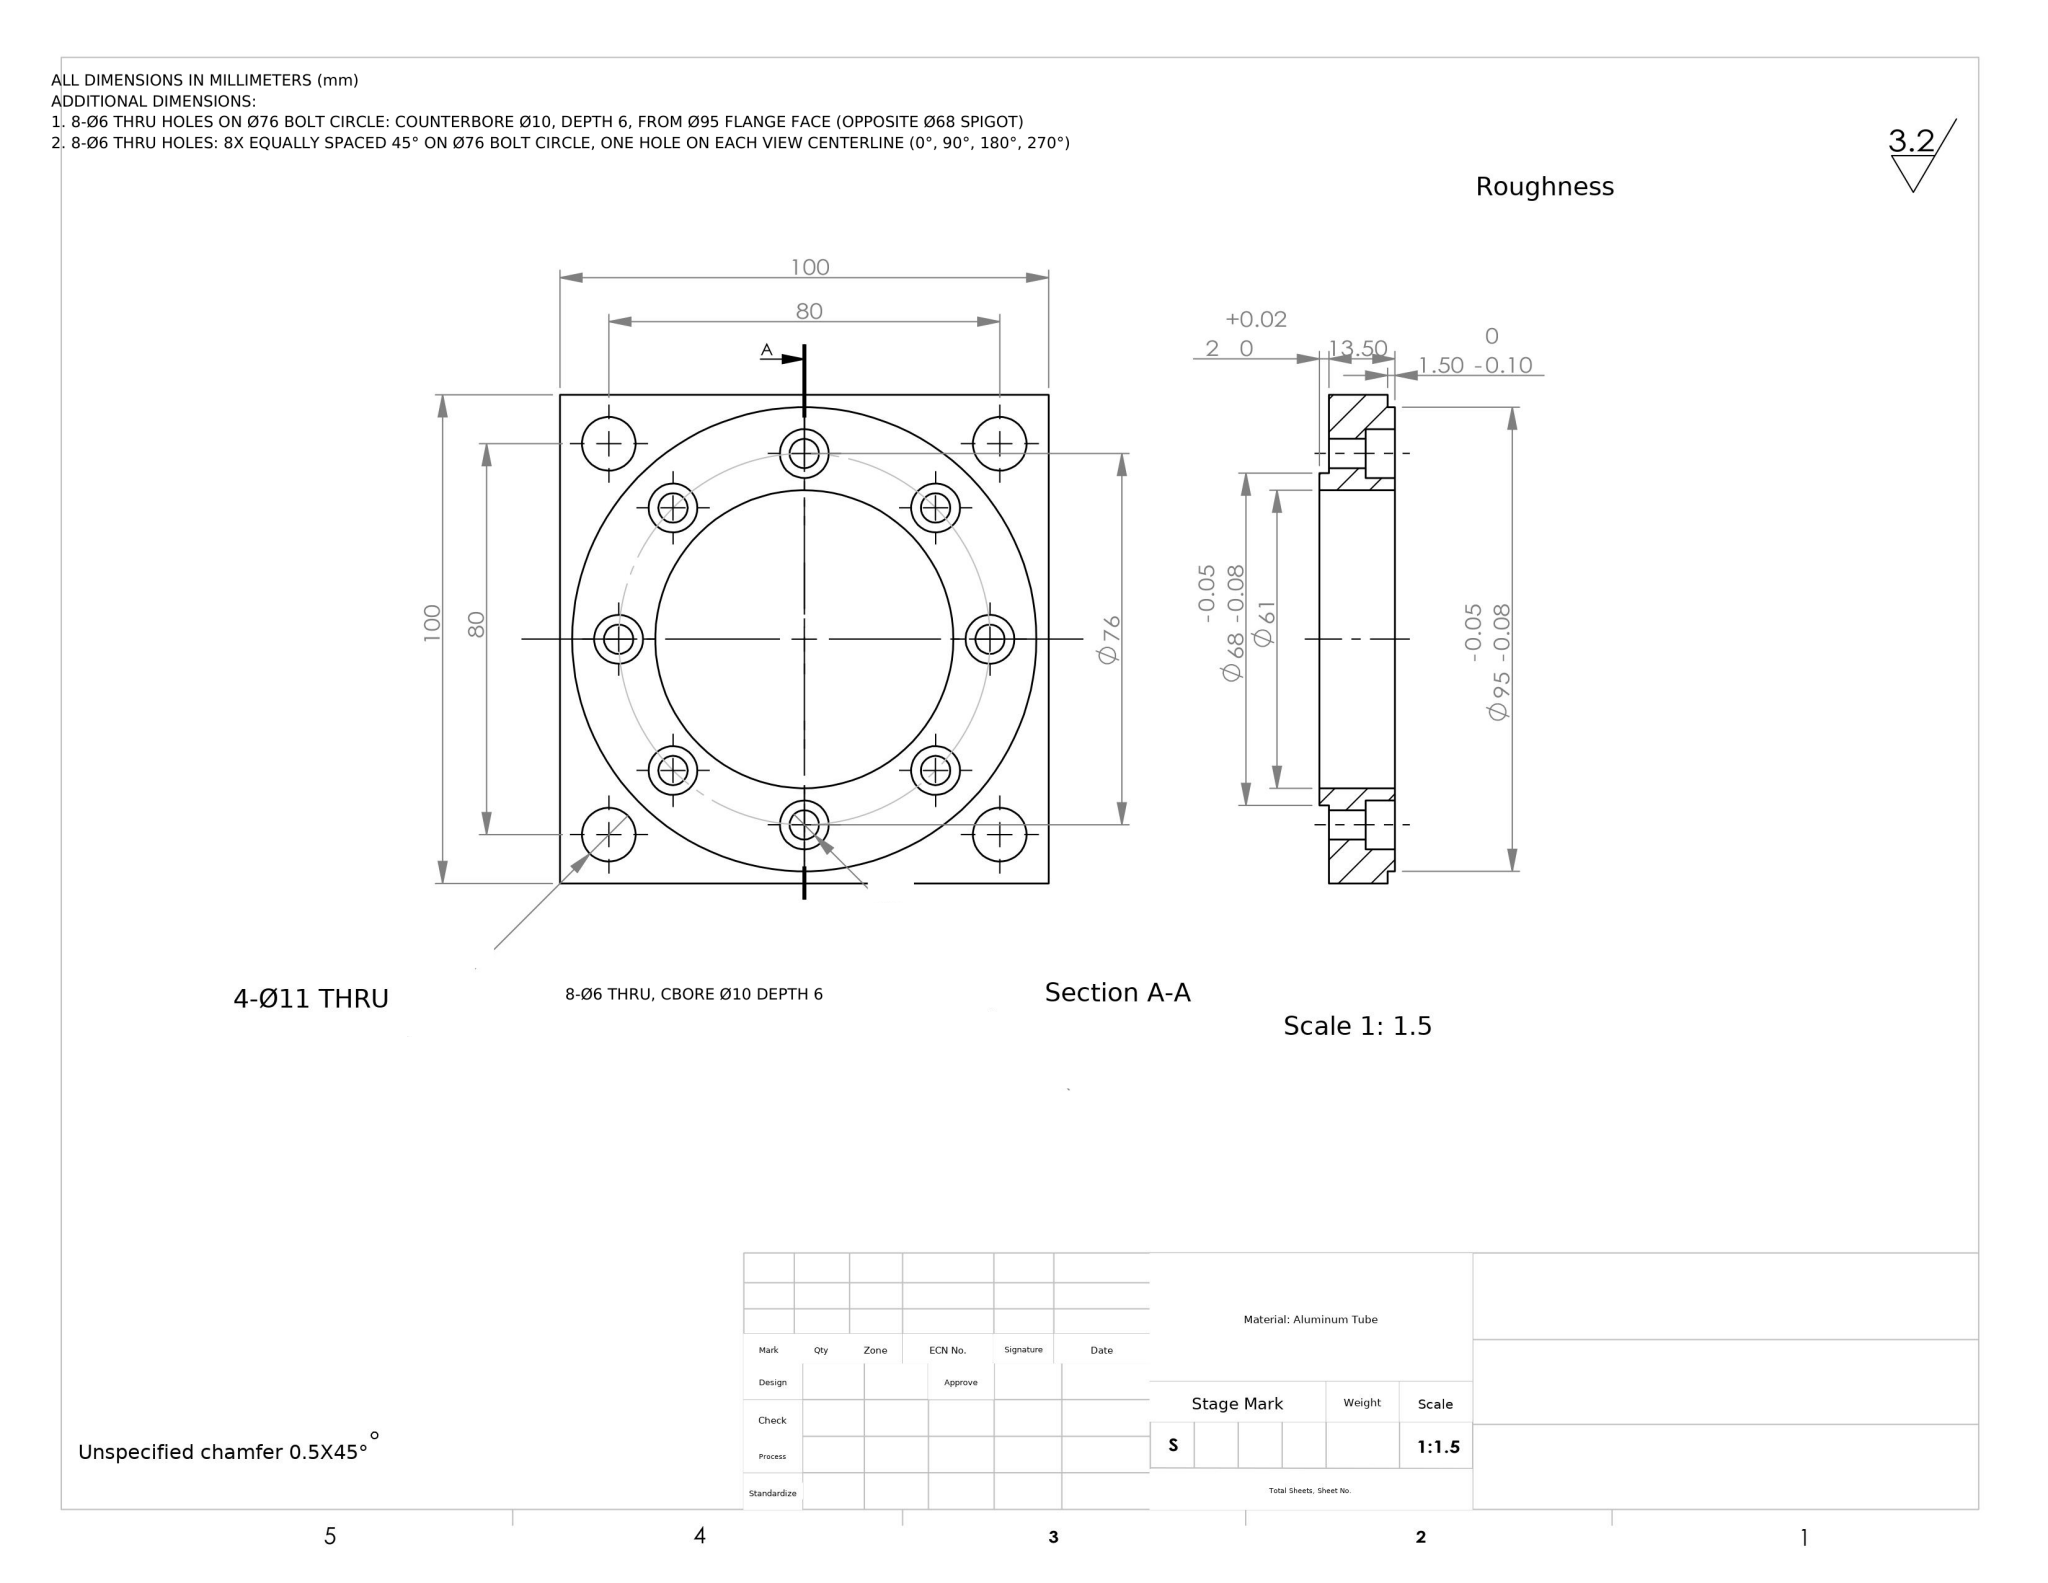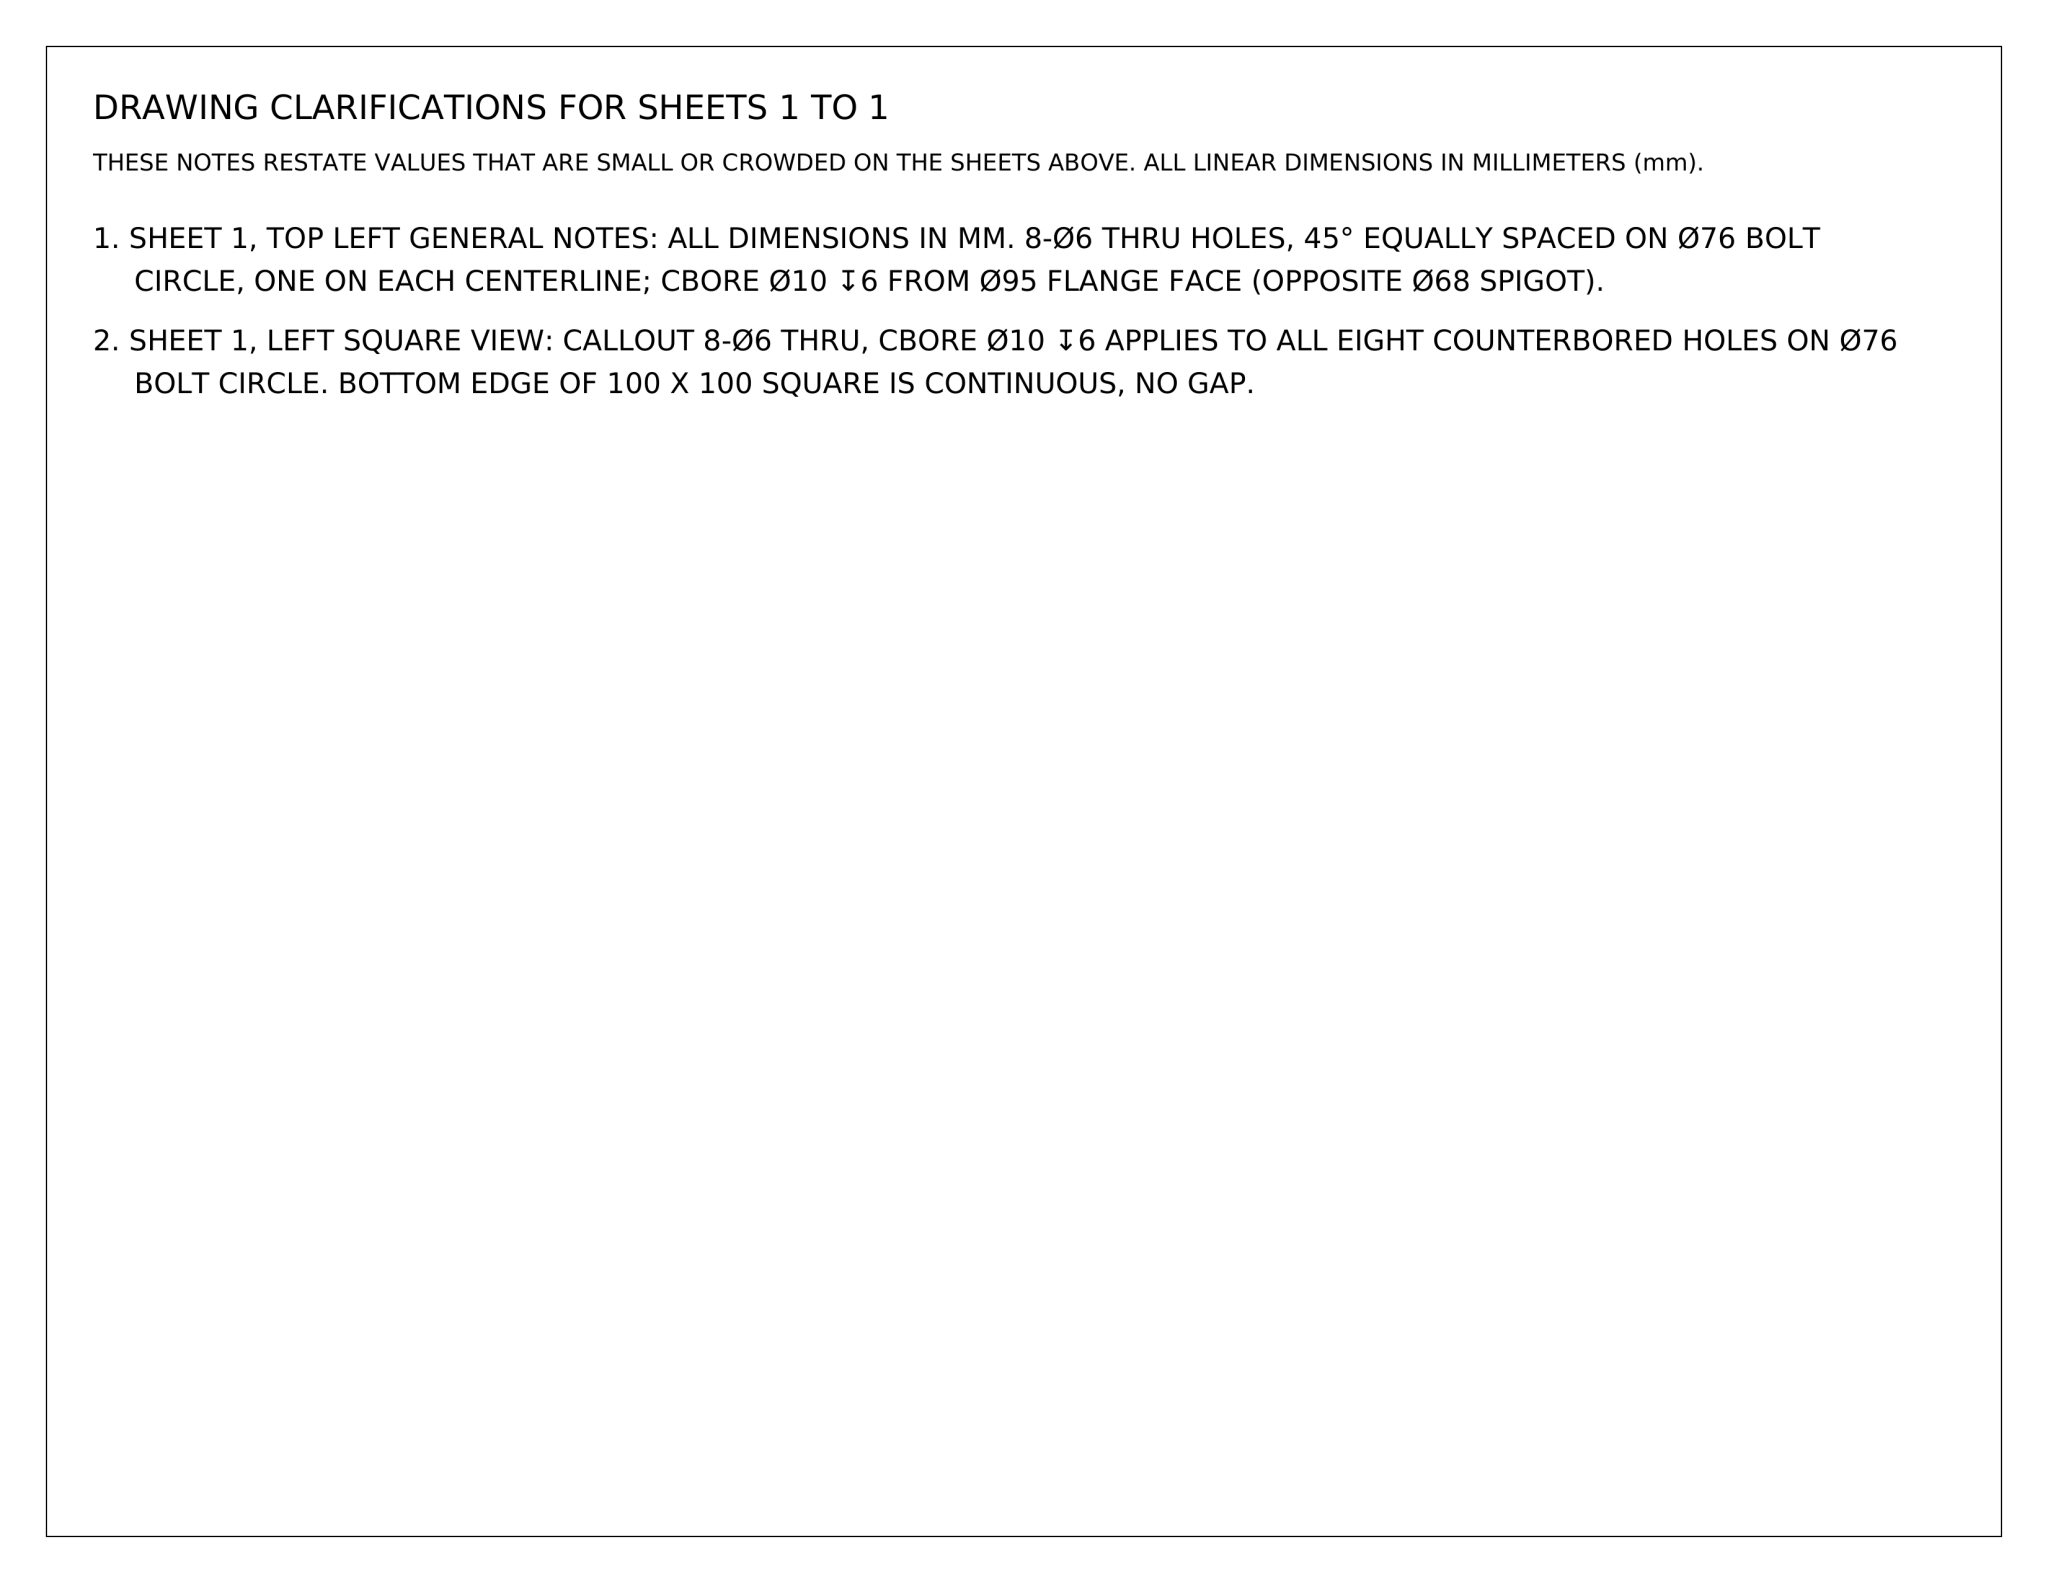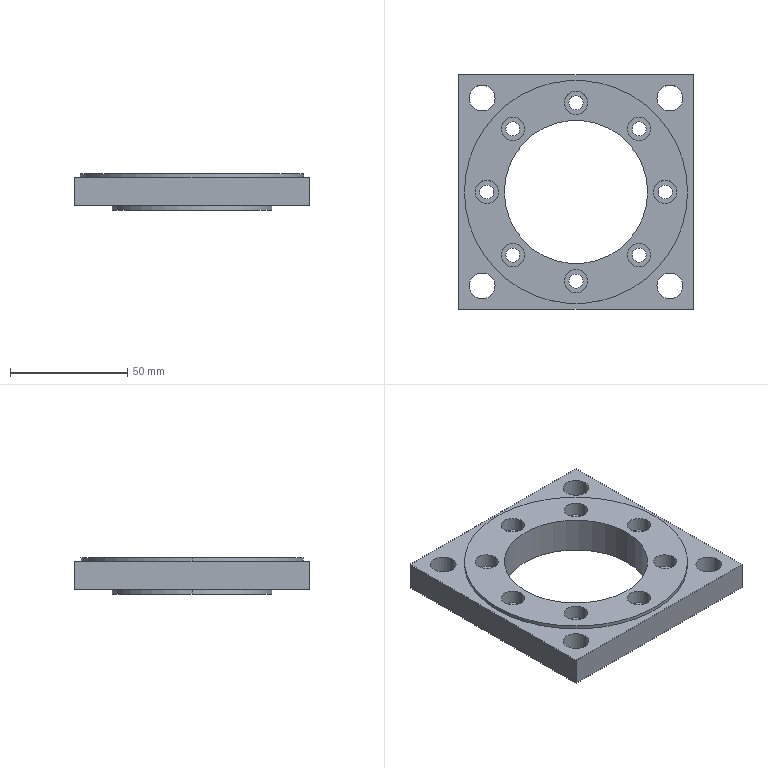Part | NX | mm | 1 solid | 62 faces | box 100 x 100 x 15.5 mm | volume 82569 mm3 | cylinder 46 | plane 16 | commonest cylinder face diameters 10 x16 6 x16 11 x8 95 x2 61 x2 68 x2